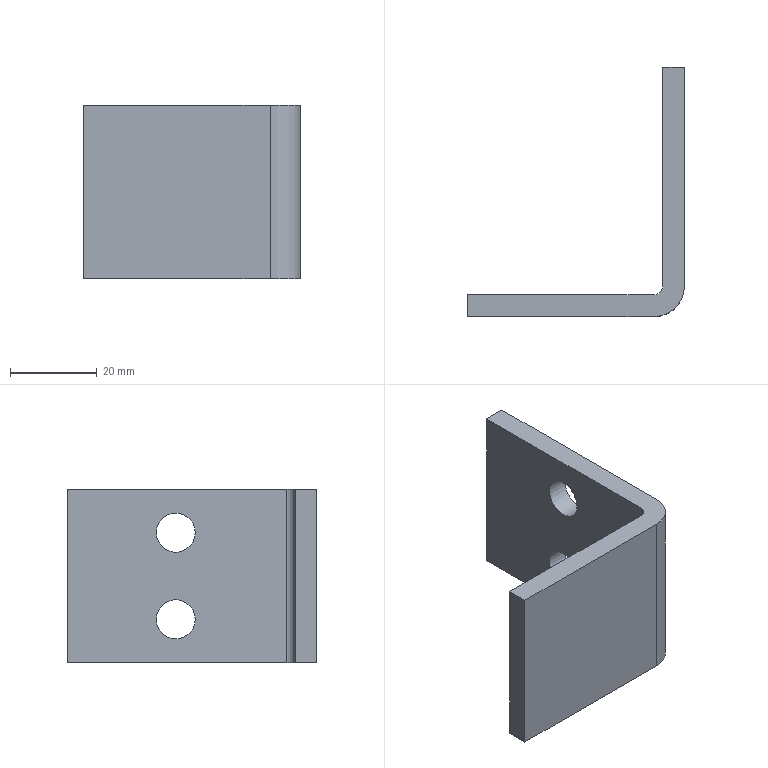Component | NX | CH3404_2-4 | 1 solid | 12 faces | box 50 x 57.5 x 40 mm | volume 19478 mm3 | plane 8 | cylinder 4 | commonest cylinder face diameters 9 x2 4 x1 14 x1
STEP:
#1=CARTESIAN_POINT('',(0.,0.,0.));
#2=DIRECTION('',(0.,0.,1.));
#3=DIRECTION('',(1.,0.,0.));
#4=AXIS2_PLACEMENT_3D('',#1,#2,#3);
#5=CARTESIAN_POINT('',(-0.,25.5,10.));
#6=VERTEX_POINT('',#5);
#7=CARTESIAN_POINT('',(0.,34.5,10.));
#8=VERTEX_POINT('',#7);
#9=CARTESIAN_POINT('',(-0.,30.,10.));
#10=DIRECTION('',(-1.,-0.,0.));
#11=DIRECTION('',(0.,-1.,0.));
#12=AXIS2_PLACEMENT_3D('',#9,#10,#11);
#13=CIRCLE('',#12,4.5);
#14=CARTESIAN_POINT('',(0.,-2.5,20.));
#15=DIRECTION('',(-1.,-0.,0.));
#16=DIRECTION('',(0.,-1.,0.));
#17=AXIS2_PLACEMENT_3D('',#14,#15,#16);
#18=PLANE('',#17);
#19=CARTESIAN_POINT('',(-32.5,-10.));
#20=DIRECTION('',(1.,0.));
#21=AXIS2_PLACEMENT_2D('',#19,#20);
#22=CIRCLE('',#21,4.5);
#23=(GEOMETRIC_REPRESENTATION_CONTEXT(2)PARAMETRIC_REPRESENTATION_CONTEXT()REPRESENTATION_CONTEXT('',''));
#24=DEFINITIONAL_REPRESENTATION('',(#22),#23);
#25=PCURVE('',#18,#24);
#26=CARTESIAN_POINT('',(-5.,30.,10.));
#27=DIRECTION('',(1.,-0.,0.));
#28=DIRECTION('',(0.,1.,0.));
#29=AXIS2_PLACEMENT_3D('',#26,#27,#28);
#30=CYLINDRICAL_SURFACE('',#29,4.5);
#31=CARTESIAN_POINT('',(3.142,5.));
#32=DIRECTION('',(-1.,0.));
#33=VECTOR('',#32,1.);
#34=LINE('',#31,#33);
#35=(GEOMETRIC_REPRESENTATION_CONTEXT(2)PARAMETRIC_REPRESENTATION_CONTEXT()REPRESENTATION_CONTEXT('',''));
#36=DEFINITIONAL_REPRESENTATION('',(#34),#35);
#37=PCURVE('',#30,#36);
#38=SURFACE_CURVE('',#13,(#25,#37),.PCURVE_S1.);
#39=EDGE_CURVE('',#6,#8,#38,.T.);
#40=ORIENTED_EDGE('',*,*,#39,.T.);
#41=CARTESIAN_POINT('',(-0.,30.,10.));
#42=DIRECTION('',(-1.,-0.,0.));
#43=DIRECTION('',(0.,-1.,0.));
#44=AXIS2_PLACEMENT_3D('',#41,#42,#43);
#45=CIRCLE('',#44,4.5);
#46=CARTESIAN_POINT('',(-32.5,-10.));
#47=DIRECTION('',(1.,0.));
#48=AXIS2_PLACEMENT_2D('',#46,#47);
#49=CIRCLE('',#48,4.5);
#50=(GEOMETRIC_REPRESENTATION_CONTEXT(2)PARAMETRIC_REPRESENTATION_CONTEXT()REPRESENTATION_CONTEXT('',''));
#51=DEFINITIONAL_REPRESENTATION('',(#49),#50);
#52=PCURVE('',#18,#51);
#53=CARTESIAN_POINT('',(9.425,5.));
#54=DIRECTION('',(-1.,0.));
#55=VECTOR('',#54,1.);
#56=LINE('',#53,#55);
#57=(GEOMETRIC_REPRESENTATION_CONTEXT(2)PARAMETRIC_REPRESENTATION_CONTEXT()REPRESENTATION_CONTEXT('',''));
#58=DEFINITIONAL_REPRESENTATION('',(#56),#57);
#59=PCURVE('',#30,#58);
#60=SURFACE_CURVE('',#45,(#52,#59),.PCURVE_S1.);
#61=EDGE_CURVE('',#8,#6,#60,.T.);
#62=ORIENTED_EDGE('',*,*,#61,.T.);
#63=EDGE_LOOP('',(#40,#62));
#64=FACE_BOUND('',#63,.T.);
#65=CARTESIAN_POINT('',(-0.,25.5,-10.));
#66=VERTEX_POINT('',#65);
#67=CARTESIAN_POINT('',(0.,34.5,-10.));
#68=VERTEX_POINT('',#67);
#69=CARTESIAN_POINT('',(-0.,30.,-10.));
#70=DIRECTION('',(-1.,-0.,0.));
#71=DIRECTION('',(0.,-1.,0.));
#72=AXIS2_PLACEMENT_3D('',#69,#70,#71);
#73=CIRCLE('',#72,4.5);
#74=CARTESIAN_POINT('',(-32.5,-30.));
#75=DIRECTION('',(1.,0.));
#76=AXIS2_PLACEMENT_2D('',#74,#75);
#77=CIRCLE('',#76,4.5);
#78=(GEOMETRIC_REPRESENTATION_CONTEXT(2)PARAMETRIC_REPRESENTATION_CONTEXT()REPRESENTATION_CONTEXT('',''));
#79=DEFINITIONAL_REPRESENTATION('',(#77),#78);
#80=PCURVE('',#18,#79);
#81=CARTESIAN_POINT('',(-5.,30.,-10.));
#82=DIRECTION('',(1.,-0.,0.));
#83=DIRECTION('',(0.,1.,0.));
#84=AXIS2_PLACEMENT_3D('',#81,#82,#83);
#85=CYLINDRICAL_SURFACE('',#84,4.5);
#86=CARTESIAN_POINT('',(3.142,5.));
#87=DIRECTION('',(-1.,0.));
#88=VECTOR('',#87,1.);
#89=LINE('',#86,#88);
#90=(GEOMETRIC_REPRESENTATION_CONTEXT(2)PARAMETRIC_REPRESENTATION_CONTEXT()REPRESENTATION_CONTEXT('',''));
#91=DEFINITIONAL_REPRESENTATION('',(#89),#90);
#92=PCURVE('',#85,#91);
#93=SURFACE_CURVE('',#73,(#80,#92),.PCURVE_S1.);
#94=EDGE_CURVE('',#66,#68,#93,.T.);
#95=ORIENTED_EDGE('',*,*,#94,.T.);
#96=CARTESIAN_POINT('',(-0.,30.,-10.));
#97=DIRECTION('',(-1.,-0.,0.));
#98=DIRECTION('',(0.,-1.,0.));
#99=AXIS2_PLACEMENT_3D('',#96,#97,#98);
#100=CIRCLE('',#99,4.5);
#101=CARTESIAN_POINT('',(-32.5,-30.));
#102=DIRECTION('',(1.,0.));
#103=AXIS2_PLACEMENT_2D('',#101,#102);
#104=CIRCLE('',#103,4.5);
#105=(GEOMETRIC_REPRESENTATION_CONTEXT(2)PARAMETRIC_REPRESENTATION_CONTEXT()REPRESENTATION_CONTEXT('',''));
#106=DEFINITIONAL_REPRESENTATION('',(#104),#105);
#107=PCURVE('',#18,#106);
#108=CARTESIAN_POINT('',(9.425,5.));
#109=DIRECTION('',(-1.,0.));
#110=VECTOR('',#109,1.);
#111=LINE('',#108,#110);
#112=(GEOMETRIC_REPRESENTATION_CONTEXT(2)PARAMETRIC_REPRESENTATION_CONTEXT()REPRESENTATION_CONTEXT('',''));
#113=DEFINITIONAL_REPRESENTATION('',(#111),#112);
#114=PCURVE('',#85,#113);
#115=SURFACE_CURVE('',#100,(#107,#114),.PCURVE_S1.);
#116=EDGE_CURVE('',#68,#66,#115,.T.);
#117=ORIENTED_EDGE('',*,*,#116,.T.);
#118=EDGE_LOOP('',(#95,#117));
#119=FACE_BOUND('',#118,.T.);
#120=CARTESIAN_POINT('',(0.,4.5,20.));
#121=VERTEX_POINT('',#120);
#122=CARTESIAN_POINT('',(-0.,55.,20.));
#123=VERTEX_POINT('',#122);
#124=CARTESIAN_POINT('',(0.,-2.5,20.));
#125=DIRECTION('',(-0.,1.,0.));
#126=VECTOR('',#125,1.);
#127=LINE('',#124,#126);
#128=CARTESIAN_POINT('',(0.,0.));
#129=DIRECTION('',(-1.,0.));
#130=VECTOR('',#129,1.);
#131=LINE('',#128,#130);
#132=(GEOMETRIC_REPRESENTATION_CONTEXT(2)PARAMETRIC_REPRESENTATION_CONTEXT()REPRESENTATION_CONTEXT('',''));
#133=DEFINITIONAL_REPRESENTATION('',(#131),#132);
#134=PCURVE('',#18,#133);
#135=CARTESIAN_POINT('',(0.,0.,20.));
#136=DIRECTION('',(0.,0.,1.));
#137=DIRECTION('',(1.,0.,0.));
#138=AXIS2_PLACEMENT_3D('',#135,#136,#137);
#139=PLANE('',#138);
#140=CARTESIAN_POINT('',(0.,-2.5));
#141=DIRECTION('',(-0.,1.));
#142=VECTOR('',#141,1.);
#143=LINE('',#140,#142);
#144=(GEOMETRIC_REPRESENTATION_CONTEXT(2)PARAMETRIC_REPRESENTATION_CONTEXT()REPRESENTATION_CONTEXT('',''));
#145=DEFINITIONAL_REPRESENTATION('',(#143),#144);
#146=PCURVE('',#139,#145);
#147=SURFACE_CURVE('',#127,(#134,#146),.PCURVE_S1.);
#148=EDGE_CURVE('',#121,#123,#147,.T.);
#149=ORIENTED_EDGE('',*,*,#148,.F.);
#150=CARTESIAN_POINT('',(0.,4.5,-20.));
#151=VERTEX_POINT('',#150);
#152=CARTESIAN_POINT('',(0.,4.5,20.));
#153=DIRECTION('',(0.,0.,-1.));
#154=VECTOR('',#153,1.);
#155=LINE('',#152,#154);
#156=CARTESIAN_POINT('',(-7.,0.));
#157=DIRECTION('',(0.,-1.));
#158=VECTOR('',#157,1.);
#159=LINE('',#156,#158);
#160=(GEOMETRIC_REPRESENTATION_CONTEXT(2)PARAMETRIC_REPRESENTATION_CONTEXT()REPRESENTATION_CONTEXT('',''));
#161=DEFINITIONAL_REPRESENTATION('',(#159),#160);
#162=PCURVE('',#18,#161);
#163=CARTESIAN_POINT('',(-7.,4.5,20.));
#164=DIRECTION('',(0.,0.,-1.));
#165=DIRECTION('',(-1.,0.,0.));
#166=AXIS2_PLACEMENT_3D('',#163,#164,#165);
#167=CYLINDRICAL_SURFACE('',#166,7.);
#168=CARTESIAN_POINT('',(3.142,0.));
#169=DIRECTION('',(0.,1.));
#170=VECTOR('',#169,1.);
#171=LINE('',#168,#170);
#172=(GEOMETRIC_REPRESENTATION_CONTEXT(2)PARAMETRIC_REPRESENTATION_CONTEXT()REPRESENTATION_CONTEXT('',''));
#173=DEFINITIONAL_REPRESENTATION('',(#171),#172);
#174=PCURVE('',#167,#173);
#175=SURFACE_CURVE('',#155,(#162,#174),.PCURVE_S1.);
#176=EDGE_CURVE('',#121,#151,#175,.T.);
#177=ORIENTED_EDGE('',*,*,#176,.T.);
#178=CARTESIAN_POINT('',(-0.,55.,-20.));
#179=VERTEX_POINT('',#178);
#180=CARTESIAN_POINT('',(0.,-2.5,-20.));
#181=DIRECTION('',(-0.,1.,0.));
#182=VECTOR('',#181,1.);
#183=LINE('',#180,#182);
#184=CARTESIAN_POINT('',(0.,-40.));
#185=DIRECTION('',(-1.,0.));
#186=VECTOR('',#185,1.);
#187=LINE('',#184,#186);
#188=(GEOMETRIC_REPRESENTATION_CONTEXT(2)PARAMETRIC_REPRESENTATION_CONTEXT()REPRESENTATION_CONTEXT('',''));
#189=DEFINITIONAL_REPRESENTATION('',(#187),#188);
#190=PCURVE('',#18,#189);
#191=CARTESIAN_POINT('',(0.,0.,-20.));
#192=DIRECTION('',(0.,0.,1.));
#193=DIRECTION('',(1.,0.,0.));
#194=AXIS2_PLACEMENT_3D('',#191,#192,#193);
#195=PLANE('',#194);
#196=CARTESIAN_POINT('',(0.,-2.5));
#197=DIRECTION('',(-0.,1.));
#198=VECTOR('',#197,1.);
#199=LINE('',#196,#198);
#200=(GEOMETRIC_REPRESENTATION_CONTEXT(2)PARAMETRIC_REPRESENTATION_CONTEXT()REPRESENTATION_CONTEXT('',''));
#201=DEFINITIONAL_REPRESENTATION('',(#199),#200);
#202=PCURVE('',#195,#201);
#203=SURFACE_CURVE('',#183,(#190,#202),.PCURVE_S1.);
#204=EDGE_CURVE('',#151,#179,#203,.T.);
#205=ORIENTED_EDGE('',*,*,#204,.T.);
#206=CARTESIAN_POINT('',(-0.,55.,20.));
#207=DIRECTION('',(0.,0.,-1.));
#208=VECTOR('',#207,1.);
#209=LINE('',#206,#208);
#210=CARTESIAN_POINT('',(-57.5,0.));
#211=DIRECTION('',(0.,-1.));
#212=VECTOR('',#211,1.);
#213=LINE('',#210,#212);
#214=(GEOMETRIC_REPRESENTATION_CONTEXT(2)PARAMETRIC_REPRESENTATION_CONTEXT()REPRESENTATION_CONTEXT('',''));
#215=DEFINITIONAL_REPRESENTATION('',(#213),#214);
#216=PCURVE('',#18,#215);
#217=CARTESIAN_POINT('',(-0.,55.,20.));
#218=DIRECTION('',(0.,-1.,0.));
#219=DIRECTION('',(1.,0.,0.));
#220=AXIS2_PLACEMENT_3D('',#217,#218,#219);
#221=PLANE('',#220);
#222=CARTESIAN_POINT('',(0.,0.));
#223=DIRECTION('',(0.,-1.));
#224=VECTOR('',#223,1.);
#225=LINE('',#222,#224);
#226=(GEOMETRIC_REPRESENTATION_CONTEXT(2)PARAMETRIC_REPRESENTATION_CONTEXT()REPRESENTATION_CONTEXT('',''));
#227=DEFINITIONAL_REPRESENTATION('',(#225),#226);
#228=PCURVE('',#221,#227);
#229=SURFACE_CURVE('',#209,(#216,#228),.PCURVE_S1.);
#230=EDGE_CURVE('',#123,#179,#229,.T.);
#231=ORIENTED_EDGE('',*,*,#230,.F.);
#232=EDGE_LOOP('',(#149,#177,#205,#231));
#233=FACE_BOUND('',#232,.T.);
#234=ADVANCED_FACE('',(#64,#119,#233),#18,.F.);
#235=CARTESIAN_POINT('',(-5.,55.,-20.));
#236=VERTEX_POINT('',#235);
#237=CARTESIAN_POINT('',(-0.,55.,-20.));
#238=DIRECTION('',(-1.,0.,0.));
#239=VECTOR('',#238,1.);
#240=LINE('',#237,#239);
#241=CARTESIAN_POINT('',(0.,-40.));
#242=DIRECTION('',(-1.,0.));
#243=VECTOR('',#242,1.);
#244=LINE('',#241,#243);
#245=(GEOMETRIC_REPRESENTATION_CONTEXT(2)PARAMETRIC_REPRESENTATION_CONTEXT()REPRESENTATION_CONTEXT('',''));
#246=DEFINITIONAL_REPRESENTATION('',(#244),#245);
#247=PCURVE('',#221,#246);
#248=CARTESIAN_POINT('',(-0.,55.));
#249=DIRECTION('',(-1.,0.));
#250=VECTOR('',#249,1.);
#251=LINE('',#248,#250);
#252=(GEOMETRIC_REPRESENTATION_CONTEXT(2)PARAMETRIC_REPRESENTATION_CONTEXT()REPRESENTATION_CONTEXT('',''));
#253=DEFINITIONAL_REPRESENTATION('',(#251),#252);
#254=PCURVE('',#195,#253);
#255=SURFACE_CURVE('',#240,(#247,#254),.PCURVE_S1.);
#256=EDGE_CURVE('',#179,#236,#255,.T.);
#257=ORIENTED_EDGE('',*,*,#256,.T.);
#258=CARTESIAN_POINT('',(-5.,55.,20.));
#259=VERTEX_POINT('',#258);
#260=CARTESIAN_POINT('',(-5.,55.,20.));
#261=DIRECTION('',(0.,0.,-1.));
#262=VECTOR('',#261,1.);
#263=LINE('',#260,#262);
#264=CARTESIAN_POINT('',(-5.,0.));
#265=DIRECTION('',(0.,-1.));
#266=VECTOR('',#265,1.);
#267=LINE('',#264,#266);
#268=(GEOMETRIC_REPRESENTATION_CONTEXT(2)PARAMETRIC_REPRESENTATION_CONTEXT()REPRESENTATION_CONTEXT('',''));
#269=DEFINITIONAL_REPRESENTATION('',(#267),#268);
#270=PCURVE('',#221,#269);
#271=CARTESIAN_POINT('',(-5.,55.,20.));
#272=DIRECTION('',(1.,0.,0.));
#273=DIRECTION('',(0.,0.,-1.));
#274=AXIS2_PLACEMENT_3D('',#271,#272,#273);
#275=PLANE('',#274);
#276=CARTESIAN_POINT('',(0.,0.));
#277=DIRECTION('',(1.,0.));
#278=VECTOR('',#277,1.);
#279=LINE('',#276,#278);
#280=(GEOMETRIC_REPRESENTATION_CONTEXT(2)PARAMETRIC_REPRESENTATION_CONTEXT()REPRESENTATION_CONTEXT('',''));
#281=DEFINITIONAL_REPRESENTATION('',(#279),#280);
#282=PCURVE('',#275,#281);
#283=SURFACE_CURVE('',#263,(#270,#282),.PCURVE_S1.);
#284=EDGE_CURVE('',#259,#236,#283,.T.);
#285=ORIENTED_EDGE('',*,*,#284,.F.);
#286=CARTESIAN_POINT('',(-0.,55.,20.));
#287=DIRECTION('',(-1.,0.,0.));
#288=VECTOR('',#287,1.);
#289=LINE('',#286,#288);
#290=CARTESIAN_POINT('',(0.,0.));
#291=DIRECTION('',(-1.,0.));
#292=VECTOR('',#291,1.);
#293=LINE('',#290,#292);
#294=(GEOMETRIC_REPRESENTATION_CONTEXT(2)PARAMETRIC_REPRESENTATION_CONTEXT()REPRESENTATION_CONTEXT('',''));
#295=DEFINITIONAL_REPRESENTATION('',(#293),#294);
#296=PCURVE('',#221,#295);
#297=CARTESIAN_POINT('',(-0.,55.));
#298=DIRECTION('',(-1.,0.));
#299=VECTOR('',#298,1.);
#300=LINE('',#297,#299);
#301=(GEOMETRIC_REPRESENTATION_CONTEXT(2)PARAMETRIC_REPRESENTATION_CONTEXT()REPRESENTATION_CONTEXT('',''));
#302=DEFINITIONAL_REPRESENTATION('',(#300),#301);
#303=PCURVE('',#139,#302);
#304=SURFACE_CURVE('',#289,(#296,#303),.PCURVE_S1.);
#305=EDGE_CURVE('',#123,#259,#304,.T.);
#306=ORIENTED_EDGE('',*,*,#305,.F.);
#307=ORIENTED_EDGE('',*,*,#230,.T.);
#308=EDGE_LOOP('',(#257,#285,#306,#307));
#309=FACE_BOUND('',#308,.T.);
#310=ADVANCED_FACE('',(#309),#221,.F.);
#311=CARTESIAN_POINT('',(-5.,34.5,10.));
#312=VERTEX_POINT('',#311);
#313=CARTESIAN_POINT('',(-5.,30.,10.));
#314=DIRECTION('',(1.,-0.,0.));
#315=DIRECTION('',(0.,1.,0.));
#316=AXIS2_PLACEMENT_3D('',#313,#314,#315);
#317=CIRCLE('',#316,4.5);
#318=CARTESIAN_POINT('',(10.,-25.));
#319=DIRECTION('',(0.,1.));
#320=AXIS2_PLACEMENT_2D('',#318,#319);
#321=CIRCLE('',#320,4.5);
#322=(GEOMETRIC_REPRESENTATION_CONTEXT(2)PARAMETRIC_REPRESENTATION_CONTEXT()REPRESENTATION_CONTEXT('',''));
#323=DEFINITIONAL_REPRESENTATION('',(#321),#322);
#324=PCURVE('',#275,#323);
#325=CARTESIAN_POINT('',(0.,0.));
#326=DIRECTION('',(1.,0.));
#327=VECTOR('',#326,1.);
#328=LINE('',#325,#327);
#329=(GEOMETRIC_REPRESENTATION_CONTEXT(2)PARAMETRIC_REPRESENTATION_CONTEXT()REPRESENTATION_CONTEXT('',''));
#330=DEFINITIONAL_REPRESENTATION('',(#328),#329);
#331=PCURVE('',#30,#330);
#332=SURFACE_CURVE('',#317,(#324,#331),.PCURVE_S1.);
#333=EDGE_CURVE('',#312,#312,#332,.T.);
#334=ORIENTED_EDGE('',*,*,#333,.T.);
#335=EDGE_LOOP('',(#334));
#336=FACE_BOUND('',#335,.T.);
#337=CARTESIAN_POINT('',(-5.,34.5,-10.));
#338=VERTEX_POINT('',#337);
#339=CARTESIAN_POINT('',(-5.,30.,-10.));
#340=DIRECTION('',(1.,-0.,0.));
#341=DIRECTION('',(0.,1.,0.));
#342=AXIS2_PLACEMENT_3D('',#339,#340,#341);
#343=CIRCLE('',#342,4.5);
#344=CARTESIAN_POINT('',(30.,-25.));
#345=DIRECTION('',(0.,1.));
#346=AXIS2_PLACEMENT_2D('',#344,#345);
#347=CIRCLE('',#346,4.5);
#348=(GEOMETRIC_REPRESENTATION_CONTEXT(2)PARAMETRIC_REPRESENTATION_CONTEXT()REPRESENTATION_CONTEXT('',''));
#349=DEFINITIONAL_REPRESENTATION('',(#347),#348);
#350=PCURVE('',#275,#349);
#351=CARTESIAN_POINT('',(0.,0.));
#352=DIRECTION('',(1.,0.));
#353=VECTOR('',#352,1.);
#354=LINE('',#351,#353);
#355=(GEOMETRIC_REPRESENTATION_CONTEXT(2)PARAMETRIC_REPRESENTATION_CONTEXT()REPRESENTATION_CONTEXT('',''));
#356=DEFINITIONAL_REPRESENTATION('',(#354),#355);
#357=PCURVE('',#85,#356);
#358=SURFACE_CURVE('',#343,(#350,#357),.PCURVE_S1.);
#359=EDGE_CURVE('',#338,#338,#358,.T.);
#360=ORIENTED_EDGE('',*,*,#359,.T.);
#361=EDGE_LOOP('',(#360));
#362=FACE_BOUND('',#361,.T.);
#363=CARTESIAN_POINT('',(-5.,4.5,-20.));
#364=VERTEX_POINT('',#363);
#365=CARTESIAN_POINT('',(-5.,55.,-20.));
#366=DIRECTION('',(0.,-1.,0.));
#367=VECTOR('',#366,1.);
#368=LINE('',#365,#367);
#369=CARTESIAN_POINT('',(40.,0.));
#370=DIRECTION('',(0.,-1.));
#371=VECTOR('',#370,1.);
#372=LINE('',#369,#371);
#373=(GEOMETRIC_REPRESENTATION_CONTEXT(2)PARAMETRIC_REPRESENTATION_CONTEXT()REPRESENTATION_CONTEXT('',''));
#374=DEFINITIONAL_REPRESENTATION('',(#372),#373);
#375=PCURVE('',#275,#374);
#376=CARTESIAN_POINT('',(-5.,55.));
#377=DIRECTION('',(0.,-1.));
#378=VECTOR('',#377,1.);
#379=LINE('',#376,#378);
#380=(GEOMETRIC_REPRESENTATION_CONTEXT(2)PARAMETRIC_REPRESENTATION_CONTEXT()REPRESENTATION_CONTEXT('',''));
#381=DEFINITIONAL_REPRESENTATION('',(#379),#380);
#382=PCURVE('',#195,#381);
#383=SURFACE_CURVE('',#368,(#375,#382),.PCURVE_S1.);
#384=EDGE_CURVE('',#236,#364,#383,.T.);
#385=ORIENTED_EDGE('',*,*,#384,.T.);
#386=CARTESIAN_POINT('',(-5.,4.5,20.));
#387=VERTEX_POINT('',#386);
#388=CARTESIAN_POINT('',(-5.,4.5,20.));
#389=DIRECTION('',(0.,0.,1.));
#390=VECTOR('',#389,1.);
#391=LINE('',#388,#390);
#392=CARTESIAN_POINT('',(0.,-50.5));
#393=DIRECTION('',(-1.,0.));
#394=VECTOR('',#393,1.);
#395=LINE('',#392,#394);
#396=(GEOMETRIC_REPRESENTATION_CONTEXT(2)PARAMETRIC_REPRESENTATION_CONTEXT()REPRESENTATION_CONTEXT('',''));
#397=DEFINITIONAL_REPRESENTATION('',(#395),#396);
#398=PCURVE('',#275,#397);
#399=CARTESIAN_POINT('',(-7.,4.5,20.));
#400=DIRECTION('',(0.,0.,1.));
#401=DIRECTION('',(1.,0.,0.));
#402=AXIS2_PLACEMENT_3D('',#399,#400,#401);
#403=CYLINDRICAL_SURFACE('',#402,2.);
#404=CARTESIAN_POINT('',(6.283,0.));
#405=DIRECTION('',(0.,1.));
#406=VECTOR('',#405,1.);
#407=LINE('',#404,#406);
#408=(GEOMETRIC_REPRESENTATION_CONTEXT(2)PARAMETRIC_REPRESENTATION_CONTEXT()REPRESENTATION_CONTEXT('',''));
#409=DEFINITIONAL_REPRESENTATION('',(#407),#408);
#410=PCURVE('',#403,#409);
#411=SURFACE_CURVE('',#391,(#398,#410),.PCURVE_S1.);
#412=EDGE_CURVE('',#364,#387,#411,.T.);
#413=ORIENTED_EDGE('',*,*,#412,.T.);
#414=CARTESIAN_POINT('',(-5.,55.,20.));
#415=DIRECTION('',(0.,-1.,0.));
#416=VECTOR('',#415,1.);
#417=LINE('',#414,#416);
#418=CARTESIAN_POINT('',(0.,0.));
#419=DIRECTION('',(0.,-1.));
#420=VECTOR('',#419,1.);
#421=LINE('',#418,#420);
#422=(GEOMETRIC_REPRESENTATION_CONTEXT(2)PARAMETRIC_REPRESENTATION_CONTEXT()REPRESENTATION_CONTEXT('',''));
#423=DEFINITIONAL_REPRESENTATION('',(#421),#422);
#424=PCURVE('',#275,#423);
#425=CARTESIAN_POINT('',(-5.,55.));
#426=DIRECTION('',(0.,-1.));
#427=VECTOR('',#426,1.);
#428=LINE('',#425,#427);
#429=(GEOMETRIC_REPRESENTATION_CONTEXT(2)PARAMETRIC_REPRESENTATION_CONTEXT()REPRESENTATION_CONTEXT('',''));
#430=DEFINITIONAL_REPRESENTATION('',(#428),#429);
#431=PCURVE('',#139,#430);
#432=SURFACE_CURVE('',#417,(#424,#431),.PCURVE_S1.);
#433=EDGE_CURVE('',#259,#387,#432,.T.);
#434=ORIENTED_EDGE('',*,*,#433,.F.);
#435=ORIENTED_EDGE('',*,*,#284,.T.);
#436=EDGE_LOOP('',(#385,#413,#434,#435));
#437=FACE_BOUND('',#436,.T.);
#438=ADVANCED_FACE('',(#336,#362,#437),#275,.F.);
#439=CARTESIAN_POINT('',(-7.,2.5,20.));
#440=VERTEX_POINT('',#439);
#441=CARTESIAN_POINT('',(-50.,2.5,20.));
#442=VERTEX_POINT('',#441);
#443=CARTESIAN_POINT('',(-5.,2.5,20.));
#444=DIRECTION('',(-1.,-0.,0.));
#445=VECTOR('',#444,1.);
#446=LINE('',#443,#445);
#447=CARTESIAN_POINT('',(-5.,2.5,20.));
#448=DIRECTION('',(0.,-1.,0.));
#449=DIRECTION('',(1.,0.,0.));
#450=AXIS2_PLACEMENT_3D('',#447,#448,#449);
#451=PLANE('',#450);
#452=CARTESIAN_POINT('',(0.,0.));
#453=DIRECTION('',(-1.,0.));
#454=VECTOR('',#453,1.);
#455=LINE('',#452,#454);
#456=(GEOMETRIC_REPRESENTATION_CONTEXT(2)PARAMETRIC_REPRESENTATION_CONTEXT()REPRESENTATION_CONTEXT('',''));
#457=DEFINITIONAL_REPRESENTATION('',(#455),#456);
#458=PCURVE('',#451,#457);
#459=CARTESIAN_POINT('',(-5.,2.5));
#460=DIRECTION('',(-1.,-0.));
#461=VECTOR('',#460,1.);
#462=LINE('',#459,#461);
#463=(GEOMETRIC_REPRESENTATION_CONTEXT(2)PARAMETRIC_REPRESENTATION_CONTEXT()REPRESENTATION_CONTEXT('',''));
#464=DEFINITIONAL_REPRESENTATION('',(#462),#463);
#465=PCURVE('',#139,#464);
#466=SURFACE_CURVE('',#446,(#458,#465),.PCURVE_S1.);
#467=EDGE_CURVE('',#440,#442,#466,.T.);
#468=ORIENTED_EDGE('',*,*,#467,.F.);
#469=CARTESIAN_POINT('',(-7.,2.5,-20.));
#470=VERTEX_POINT('',#469);
#471=CARTESIAN_POINT('',(-7.,2.5,-20.));
#472=DIRECTION('',(0.,0.,-1.));
#473=VECTOR('',#472,1.);
#474=LINE('',#471,#473);
#475=CARTESIAN_POINT('',(-2.,-40.));
#476=DIRECTION('',(0.,-1.));
#477=VECTOR('',#476,1.);
#478=LINE('',#475,#477);
#479=(GEOMETRIC_REPRESENTATION_CONTEXT(2)PARAMETRIC_REPRESENTATION_CONTEXT()REPRESENTATION_CONTEXT('',''));
#480=DEFINITIONAL_REPRESENTATION('',(#478),#479);
#481=PCURVE('',#451,#480);
#482=CARTESIAN_POINT('',(4.712,-40.));
#483=DIRECTION('',(0.,-1.));
#484=VECTOR('',#483,1.);
#485=LINE('',#482,#484);
#486=(GEOMETRIC_REPRESENTATION_CONTEXT(2)PARAMETRIC_REPRESENTATION_CONTEXT()REPRESENTATION_CONTEXT('',''));
#487=DEFINITIONAL_REPRESENTATION('',(#485),#486);
#488=PCURVE('',#403,#487);
#489=SURFACE_CURVE('',#474,(#481,#488),.PCURVE_S1.);
#490=EDGE_CURVE('',#440,#470,#489,.T.);
#491=ORIENTED_EDGE('',*,*,#490,.T.);
#492=CARTESIAN_POINT('',(-50.,2.5,-20.));
#493=VERTEX_POINT('',#492);
#494=CARTESIAN_POINT('',(-5.,2.5,-20.));
#495=DIRECTION('',(-1.,-0.,0.));
#496=VECTOR('',#495,1.);
#497=LINE('',#494,#496);
#498=CARTESIAN_POINT('',(0.,-40.));
#499=DIRECTION('',(-1.,0.));
#500=VECTOR('',#499,1.);
#501=LINE('',#498,#500);
#502=(GEOMETRIC_REPRESENTATION_CONTEXT(2)PARAMETRIC_REPRESENTATION_CONTEXT()REPRESENTATION_CONTEXT('',''));
#503=DEFINITIONAL_REPRESENTATION('',(#501),#502);
#504=PCURVE('',#451,#503);
#505=CARTESIAN_POINT('',(-5.,2.5));
#506=DIRECTION('',(-1.,-0.));
#507=VECTOR('',#506,1.);
#508=LINE('',#505,#507);
#509=(GEOMETRIC_REPRESENTATION_CONTEXT(2)PARAMETRIC_REPRESENTATION_CONTEXT()REPRESENTATION_CONTEXT('',''));
#510=DEFINITIONAL_REPRESENTATION('',(#508),#509);
#511=PCURVE('',#195,#510);
#512=SURFACE_CURVE('',#497,(#504,#511),.PCURVE_S1.);
#513=EDGE_CURVE('',#470,#493,#512,.T.);
#514=ORIENTED_EDGE('',*,*,#513,.T.);
#515=CARTESIAN_POINT('',(-50.,2.5,20.));
#516=DIRECTION('',(0.,0.,-1.));
#517=VECTOR('',#516,1.);
#518=LINE('',#515,#517);
#519=CARTESIAN_POINT('',(-45.,0.));
#520=DIRECTION('',(0.,-1.));
#521=VECTOR('',#520,1.);
#522=LINE('',#519,#521);
#523=(GEOMETRIC_REPRESENTATION_CONTEXT(2)PARAMETRIC_REPRESENTATION_CONTEXT()REPRESENTATION_CONTEXT('',''));
#524=DEFINITIONAL_REPRESENTATION('',(#522),#523);
#525=PCURVE('',#451,#524);
#526=CARTESIAN_POINT('',(-50.,2.5,20.));
#527=DIRECTION('',(1.,0.,0.));
#528=DIRECTION('',(0.,0.,-1.));
#529=AXIS2_PLACEMENT_3D('',#526,#527,#528);
#530=PLANE('',#529);
#531=CARTESIAN_POINT('',(0.,0.));
#532=DIRECTION('',(1.,0.));
#533=VECTOR('',#532,1.);
#534=LINE('',#531,#533);
#535=(GEOMETRIC_REPRESENTATION_CONTEXT(2)PARAMETRIC_REPRESENTATION_CONTEXT()REPRESENTATION_CONTEXT('',''));
#536=DEFINITIONAL_REPRESENTATION('',(#534),#535);
#537=PCURVE('',#530,#536);
#538=SURFACE_CURVE('',#518,(#525,#537),.PCURVE_S1.);
#539=EDGE_CURVE('',#442,#493,#538,.T.);
#540=ORIENTED_EDGE('',*,*,#539,.F.);
#541=EDGE_LOOP('',(#468,#491,#514,#540));
#542=FACE_BOUND('',#541,.T.);
#543=ADVANCED_FACE('',(#542),#451,.F.);
#544=CARTESIAN_POINT('',(-50.,-2.5,-20.));
#545=VERTEX_POINT('',#544);
#546=CARTESIAN_POINT('',(-50.,2.5,-20.));
#547=DIRECTION('',(0.,-1.,0.));
#548=VECTOR('',#547,1.);
#549=LINE('',#546,#548);
#550=CARTESIAN_POINT('',(40.,0.));
#551=DIRECTION('',(0.,-1.));
#552=VECTOR('',#551,1.);
#553=LINE('',#550,#552);
#554=(GEOMETRIC_REPRESENTATION_CONTEXT(2)PARAMETRIC_REPRESENTATION_CONTEXT()REPRESENTATION_CONTEXT('',''));
#555=DEFINITIONAL_REPRESENTATION('',(#553),#554);
#556=PCURVE('',#530,#555);
#557=CARTESIAN_POINT('',(-50.,2.5));
#558=DIRECTION('',(0.,-1.));
#559=VECTOR('',#558,1.);
#560=LINE('',#557,#559);
#561=(GEOMETRIC_REPRESENTATION_CONTEXT(2)PARAMETRIC_REPRESENTATION_CONTEXT()REPRESENTATION_CONTEXT('',''));
#562=DEFINITIONAL_REPRESENTATION('',(#560),#561);
#563=PCURVE('',#195,#562);
#564=SURFACE_CURVE('',#549,(#556,#563),.PCURVE_S1.);
#565=EDGE_CURVE('',#493,#545,#564,.T.);
#566=ORIENTED_EDGE('',*,*,#565,.T.);
#567=CARTESIAN_POINT('',(-50.,-2.5,20.));
#568=VERTEX_POINT('',#567);
#569=CARTESIAN_POINT('',(-50.,-2.5,20.));
#570=DIRECTION('',(0.,0.,-1.));
#571=VECTOR('',#570,1.);
#572=LINE('',#569,#571);
#573=CARTESIAN_POINT('',(0.,-5.));
#574=DIRECTION('',(1.,0.));
#575=VECTOR('',#574,1.);
#576=LINE('',#573,#575);
#577=(GEOMETRIC_REPRESENTATION_CONTEXT(2)PARAMETRIC_REPRESENTATION_CONTEXT()REPRESENTATION_CONTEXT('',''));
#578=DEFINITIONAL_REPRESENTATION('',(#576),#577);
#579=PCURVE('',#530,#578);
#580=CARTESIAN_POINT('',(-50.,-2.5,20.));
#581=DIRECTION('',(-0.,1.,0.));
#582=DIRECTION('',(-1.,-0.,0.));
#583=AXIS2_PLACEMENT_3D('',#580,#581,#582);
#584=PLANE('',#583);
#585=CARTESIAN_POINT('',(0.,0.));
#586=DIRECTION('',(0.,-1.));
#587=VECTOR('',#586,1.);
#588=LINE('',#585,#587);
#589=(GEOMETRIC_REPRESENTATION_CONTEXT(2)PARAMETRIC_REPRESENTATION_CONTEXT()REPRESENTATION_CONTEXT('',''));
#590=DEFINITIONAL_REPRESENTATION('',(#588),#589);
#591=PCURVE('',#584,#590);
#592=SURFACE_CURVE('',#572,(#579,#591),.PCURVE_S1.);
#593=EDGE_CURVE('',#568,#545,#592,.T.);
#594=ORIENTED_EDGE('',*,*,#593,.F.);
#595=CARTESIAN_POINT('',(-50.,2.5,20.));
#596=DIRECTION('',(0.,-1.,0.));
#597=VECTOR('',#596,1.);
#598=LINE('',#595,#597);
#599=CARTESIAN_POINT('',(0.,0.));
#600=DIRECTION('',(0.,-1.));
#601=VECTOR('',#600,1.);
#602=LINE('',#599,#601);
#603=(GEOMETRIC_REPRESENTATION_CONTEXT(2)PARAMETRIC_REPRESENTATION_CONTEXT()REPRESENTATION_CONTEXT('',''));
#604=DEFINITIONAL_REPRESENTATION('',(#602),#603);
#605=PCURVE('',#530,#604);
#606=CARTESIAN_POINT('',(-50.,2.5));
#607=DIRECTION('',(0.,-1.));
#608=VECTOR('',#607,1.);
#609=LINE('',#606,#608);
#610=(GEOMETRIC_REPRESENTATION_CONTEXT(2)PARAMETRIC_REPRESENTATION_CONTEXT()REPRESENTATION_CONTEXT('',''));
#611=DEFINITIONAL_REPRESENTATION('',(#609),#610);
#612=PCURVE('',#139,#611);
#613=SURFACE_CURVE('',#598,(#605,#612),.PCURVE_S1.);
#614=EDGE_CURVE('',#442,#568,#613,.T.);
#615=ORIENTED_EDGE('',*,*,#614,.F.);
#616=ORIENTED_EDGE('',*,*,#539,.T.);
#617=EDGE_LOOP('',(#566,#594,#615,#616));
#618=FACE_BOUND('',#617,.T.);
#619=ADVANCED_FACE('',(#618),#530,.F.);
#620=CARTESIAN_POINT('',(-7.,-2.5,-20.));
#621=VERTEX_POINT('',#620);
#622=CARTESIAN_POINT('',(-50.,-2.5,-20.));
#623=DIRECTION('',(1.,0.,0.));
#624=VECTOR('',#623,1.);
#625=LINE('',#622,#624);
#626=CARTESIAN_POINT('',(0.,-40.));
#627=DIRECTION('',(-1.,0.));
#628=VECTOR('',#627,1.);
#629=LINE('',#626,#628);
#630=(GEOMETRIC_REPRESENTATION_CONTEXT(2)PARAMETRIC_REPRESENTATION_CONTEXT()REPRESENTATION_CONTEXT('',''));
#631=DEFINITIONAL_REPRESENTATION('',(#629),#630);
#632=PCURVE('',#584,#631);
#633=CARTESIAN_POINT('',(-50.,-2.5));
#634=DIRECTION('',(1.,0.));
#635=VECTOR('',#634,1.);
#636=LINE('',#633,#635);
#637=(GEOMETRIC_REPRESENTATION_CONTEXT(2)PARAMETRIC_REPRESENTATION_CONTEXT()REPRESENTATION_CONTEXT('',''));
#638=DEFINITIONAL_REPRESENTATION('',(#636),#637);
#639=PCURVE('',#195,#638);
#640=SURFACE_CURVE('',#625,(#632,#639),.PCURVE_S1.);
#641=EDGE_CURVE('',#545,#621,#640,.T.);
#642=ORIENTED_EDGE('',*,*,#641,.T.);
#643=CARTESIAN_POINT('',(-7.,-2.5,20.));
#644=VERTEX_POINT('',#643);
#645=CARTESIAN_POINT('',(-7.,-2.5,20.));
#646=DIRECTION('',(0.,0.,1.));
#647=VECTOR('',#646,1.);
#648=LINE('',#645,#647);
#649=CARTESIAN_POINT('',(-43.,0.));
#650=DIRECTION('',(0.,1.));
#651=VECTOR('',#650,1.);
#652=LINE('',#649,#651);
#653=(GEOMETRIC_REPRESENTATION_CONTEXT(2)PARAMETRIC_REPRESENTATION_CONTEXT()REPRESENTATION_CONTEXT('',''));
#654=DEFINITIONAL_REPRESENTATION('',(#652),#653);
#655=PCURVE('',#584,#654);
#656=CARTESIAN_POINT('',(4.712,0.));
#657=DIRECTION('',(0.,-1.));
#658=VECTOR('',#657,1.);
#659=LINE('',#656,#658);
#660=(GEOMETRIC_REPRESENTATION_CONTEXT(2)PARAMETRIC_REPRESENTATION_CONTEXT()REPRESENTATION_CONTEXT('',''));
#661=DEFINITIONAL_REPRESENTATION('',(#659),#660);
#662=PCURVE('',#167,#661);
#663=SURFACE_CURVE('',#648,(#655,#662),.PCURVE_S1.);
#664=EDGE_CURVE('',#621,#644,#663,.T.);
#665=ORIENTED_EDGE('',*,*,#664,.T.);
#666=CARTESIAN_POINT('',(-50.,-2.5,20.));
#667=DIRECTION('',(1.,0.,0.));
#668=VECTOR('',#667,1.);
#669=LINE('',#666,#668);
#670=CARTESIAN_POINT('',(0.,0.));
#671=DIRECTION('',(-1.,0.));
#672=VECTOR('',#671,1.);
#673=LINE('',#670,#672);
#674=(GEOMETRIC_REPRESENTATION_CONTEXT(2)PARAMETRIC_REPRESENTATION_CONTEXT()REPRESENTATION_CONTEXT('',''));
#675=DEFINITIONAL_REPRESENTATION('',(#673),#674);
#676=PCURVE('',#584,#675);
#677=CARTESIAN_POINT('',(-50.,-2.5));
#678=DIRECTION('',(1.,0.));
#679=VECTOR('',#678,1.);
#680=LINE('',#677,#679);
#681=(GEOMETRIC_REPRESENTATION_CONTEXT(2)PARAMETRIC_REPRESENTATION_CONTEXT()REPRESENTATION_CONTEXT('',''));
#682=DEFINITIONAL_REPRESENTATION('',(#680),#681);
#683=PCURVE('',#139,#682);
#684=SURFACE_CURVE('',#669,(#676,#683),.PCURVE_S1.);
#685=EDGE_CURVE('',#568,#644,#684,.T.);
#686=ORIENTED_EDGE('',*,*,#685,.F.);
#687=ORIENTED_EDGE('',*,*,#593,.T.);
#688=EDGE_LOOP('',(#642,#665,#686,#687));
#689=FACE_BOUND('',#688,.T.);
#690=ADVANCED_FACE('',(#689),#584,.F.);
#691=ORIENTED_EDGE('',*,*,#685,.T.);
#692=CARTESIAN_POINT('',(-7.,4.5,20.));
#693=DIRECTION('',(0.,0.,1.));
#694=DIRECTION('',(1.,0.,0.));
#695=AXIS2_PLACEMENT_3D('',#692,#693,#694);
#696=CIRCLE('',#695,7.);
#697=CARTESIAN_POINT('',(-7.,4.5));
#698=DIRECTION('',(1.,0.));
#699=AXIS2_PLACEMENT_2D('',#697,#698);
#700=CIRCLE('',#699,7.);
#701=(GEOMETRIC_REPRESENTATION_CONTEXT(2)PARAMETRIC_REPRESENTATION_CONTEXT()REPRESENTATION_CONTEXT('',''));
#702=DEFINITIONAL_REPRESENTATION('',(#700),#701);
#703=PCURVE('',#139,#702);
#704=CARTESIAN_POINT('',(9.425,0.));
#705=DIRECTION('',(-1.,0.));
#706=VECTOR('',#705,1.);
#707=LINE('',#704,#706);
#708=(GEOMETRIC_REPRESENTATION_CONTEXT(2)PARAMETRIC_REPRESENTATION_CONTEXT()REPRESENTATION_CONTEXT('',''));
#709=DEFINITIONAL_REPRESENTATION('',(#707),#708);
#710=PCURVE('',#167,#709);
#711=SURFACE_CURVE('',#696,(#703,#710),.PCURVE_S1.);
#712=EDGE_CURVE('',#644,#121,#711,.T.);
#713=ORIENTED_EDGE('',*,*,#712,.T.);
#714=ORIENTED_EDGE('',*,*,#148,.T.);
#715=ORIENTED_EDGE('',*,*,#305,.T.);
#716=ORIENTED_EDGE('',*,*,#433,.T.);
#717=CARTESIAN_POINT('',(-7.,4.5,20.));
#718=DIRECTION('',(0.,0.,-1.));
#719=DIRECTION('',(1.,0.,0.));
#720=AXIS2_PLACEMENT_3D('',#717,#718,#719);
#721=CIRCLE('',#720,2.);
#722=CARTESIAN_POINT('',(-5.,4.5));
#723=CARTESIAN_POINT('',(-5.,1.036));
#724=CARTESIAN_POINT('',(-8.,2.768));
#725=CARTESIAN_POINT('',(-11.,4.5));
#726=CARTESIAN_POINT('',(-8.,6.232));
#727=CARTESIAN_POINT('',(-5.,7.964));
#728=CARTESIAN_POINT('',(-5.,4.5));
#729=(BOUNDED_CURVE()B_SPLINE_CURVE(2,(#722,#723,#724,#725,#726,#727,#728),.UNSPECIFIED.,.T.,.F.)B_SPLINE_CURVE_WITH_KNOTS((1,2,2,2,2,1),(-2.094,0.,2.094,4.189,6.283,8.378),.UNSPECIFIED.)CURVE()GEOMETRIC_REPRESENTATION_ITEM()RATIONAL_B_SPLINE_CURVE((1.,0.5,1.,0.5,1.,0.5,1.))REPRESENTATION_ITEM(''));
#730=(GEOMETRIC_REPRESENTATION_CONTEXT(2)PARAMETRIC_REPRESENTATION_CONTEXT()REPRESENTATION_CONTEXT('',''));
#731=DEFINITIONAL_REPRESENTATION('',(#729),#730);
#732=PCURVE('',#139,#731);
#733=CARTESIAN_POINT('',(6.283,0.));
#734=DIRECTION('',(-1.,0.));
#735=VECTOR('',#734,1.);
#736=LINE('',#733,#735);
#737=(GEOMETRIC_REPRESENTATION_CONTEXT(2)PARAMETRIC_REPRESENTATION_CONTEXT()REPRESENTATION_CONTEXT('',''));
#738=DEFINITIONAL_REPRESENTATION('',(#736),#737);
#739=PCURVE('',#403,#738);
#740=SURFACE_CURVE('',#721,(#732,#739),.PCURVE_S1.);
#741=EDGE_CURVE('',#387,#440,#740,.T.);
#742=ORIENTED_EDGE('',*,*,#741,.T.);
#743=ORIENTED_EDGE('',*,*,#467,.T.);
#744=ORIENTED_EDGE('',*,*,#614,.T.);
#745=EDGE_LOOP('',(#691,#713,#714,#715,#716,#742,#743,#744));
#746=FACE_BOUND('',#745,.T.);
#747=ADVANCED_FACE('',(#746),#139,.T.);
#748=ORIENTED_EDGE('',*,*,#204,.F.);
#749=CARTESIAN_POINT('',(-7.,4.5,-20.));
#750=DIRECTION('',(0.,0.,-1.));
#751=DIRECTION('',(1.,0.,0.));
#752=AXIS2_PLACEMENT_3D('',#749,#750,#751);
#753=CIRCLE('',#752,7.);
#754=CARTESIAN_POINT('',(0.,4.5));
#755=CARTESIAN_POINT('',(0.,-7.624));
#756=CARTESIAN_POINT('',(-10.5,-1.562));
#757=CARTESIAN_POINT('',(-21.,4.5));
#758=CARTESIAN_POINT('',(-10.5,10.562));
#759=CARTESIAN_POINT('',(-0.,16.624));
#760=CARTESIAN_POINT('',(0.,4.5));
#761=(BOUNDED_CURVE()B_SPLINE_CURVE(2,(#754,#755,#756,#757,#758,#759,#760),.UNSPECIFIED.,.T.,.F.)B_SPLINE_CURVE_WITH_KNOTS((1,2,2,2,2,1),(-2.094,0.,2.094,4.189,6.283,8.378),.UNSPECIFIED.)CURVE()GEOMETRIC_REPRESENTATION_ITEM()RATIONAL_B_SPLINE_CURVE((1.,0.5,1.,0.5,1.,0.5,1.))REPRESENTATION_ITEM(''));
#762=(GEOMETRIC_REPRESENTATION_CONTEXT(2)PARAMETRIC_REPRESENTATION_CONTEXT()REPRESENTATION_CONTEXT('',''));
#763=DEFINITIONAL_REPRESENTATION('',(#761),#762);
#764=PCURVE('',#195,#763);
#765=CARTESIAN_POINT('',(3.142,40.));
#766=DIRECTION('',(1.,0.));
#767=VECTOR('',#766,1.);
#768=LINE('',#765,#767);
#769=(GEOMETRIC_REPRESENTATION_CONTEXT(2)PARAMETRIC_REPRESENTATION_CONTEXT()REPRESENTATION_CONTEXT('',''));
#770=DEFINITIONAL_REPRESENTATION('',(#768),#769);
#771=PCURVE('',#167,#770);
#772=SURFACE_CURVE('',#753,(#764,#771),.PCURVE_S1.);
#773=EDGE_CURVE('',#151,#621,#772,.T.);
#774=ORIENTED_EDGE('',*,*,#773,.T.);
#775=ORIENTED_EDGE('',*,*,#641,.F.);
#776=ORIENTED_EDGE('',*,*,#565,.F.);
#777=ORIENTED_EDGE('',*,*,#513,.F.);
#778=CARTESIAN_POINT('',(-7.,4.5,-20.));
#779=DIRECTION('',(0.,0.,1.));
#780=DIRECTION('',(1.,0.,0.));
#781=AXIS2_PLACEMENT_3D('',#778,#779,#780);
#782=CIRCLE('',#781,2.);
#783=CARTESIAN_POINT('',(-7.,4.5));
#784=DIRECTION('',(1.,0.));
#785=AXIS2_PLACEMENT_2D('',#783,#784);
#786=CIRCLE('',#785,2.);
#787=(GEOMETRIC_REPRESENTATION_CONTEXT(2)PARAMETRIC_REPRESENTATION_CONTEXT()REPRESENTATION_CONTEXT('',''));
#788=DEFINITIONAL_REPRESENTATION('',(#786),#787);
#789=PCURVE('',#195,#788);
#790=CARTESIAN_POINT('',(0.,-40.));
#791=DIRECTION('',(1.,0.));
#792=VECTOR('',#791,1.);
#793=LINE('',#790,#792);
#794=(GEOMETRIC_REPRESENTATION_CONTEXT(2)PARAMETRIC_REPRESENTATION_CONTEXT()REPRESENTATION_CONTEXT('',''));
#795=DEFINITIONAL_REPRESENTATION('',(#793),#794);
#796=PCURVE('',#403,#795);
#797=SURFACE_CURVE('',#782,(#789,#796),.PCURVE_S1.);
#798=EDGE_CURVE('',#470,#364,#797,.T.);
#799=ORIENTED_EDGE('',*,*,#798,.T.);
#800=ORIENTED_EDGE('',*,*,#384,.F.);
#801=ORIENTED_EDGE('',*,*,#256,.F.);
#802=EDGE_LOOP('',(#748,#774,#775,#776,#777,#799,#800,#801));
#803=FACE_BOUND('',#802,.T.);
#804=ADVANCED_FACE('',(#803),#195,.F.);
#805=ORIENTED_EDGE('',*,*,#359,.T.);
#806=CARTESIAN_POINT('',(-5.,34.5,-10.));
#807=CARTESIAN_POINT('',(0.,34.5,-10.));
#808=B_SPLINE_CURVE_WITH_KNOTS('',1,(#806,#807),.UNSPECIFIED.,.F.,.F.,(2,2),(0.,5.),.PIECEWISE_BEZIER_KNOTS.);
#809=CARTESIAN_POINT('',(6.283,0.));
#810=DIRECTION('',(0.,1.));
#811=VECTOR('',#810,1.);
#812=LINE('',#809,#811);
#813=(GEOMETRIC_REPRESENTATION_CONTEXT(2)PARAMETRIC_REPRESENTATION_CONTEXT()REPRESENTATION_CONTEXT('',''));
#814=DEFINITIONAL_REPRESENTATION('',(#812),#813);
#815=PCURVE('',#85,#814);
#816=CARTESIAN_POINT('',(0.,0.));
#817=DIRECTION('',(0.,1.));
#818=VECTOR('',#817,1.);
#819=LINE('',#816,#818);
#820=(GEOMETRIC_REPRESENTATION_CONTEXT(2)PARAMETRIC_REPRESENTATION_CONTEXT()REPRESENTATION_CONTEXT('',''));
#821=DEFINITIONAL_REPRESENTATION('',(#819),#820);
#822=PCURVE('',#85,#821);
#823=SEAM_CURVE('',#808,(#815,#822),.PCURVE_S1.);
#824=EDGE_CURVE('',#338,#68,#823,.T.);
#825=ORIENTED_EDGE('',*,*,#824,.T.);
#826=ORIENTED_EDGE('',*,*,#116,.T.);
#827=ORIENTED_EDGE('',*,*,#94,.T.);
#828=ORIENTED_EDGE('',*,*,#824,.F.);
#829=EDGE_LOOP('',(#805,#825,#826,#827,#828));
#830=FACE_BOUND('',#829,.F.);
#831=ADVANCED_FACE('',(#830),#85,.F.);
#832=ORIENTED_EDGE('',*,*,#333,.T.);
#833=CARTESIAN_POINT('',(-5.,34.5,10.));
#834=CARTESIAN_POINT('',(0.,34.5,10.));
#835=B_SPLINE_CURVE_WITH_KNOTS('',1,(#833,#834),.UNSPECIFIED.,.F.,.F.,(2,2),(0.,5.),.PIECEWISE_BEZIER_KNOTS.);
#836=CARTESIAN_POINT('',(6.283,0.));
#837=DIRECTION('',(0.,1.));
#838=VECTOR('',#837,1.);
#839=LINE('',#836,#838);
#840=(GEOMETRIC_REPRESENTATION_CONTEXT(2)PARAMETRIC_REPRESENTATION_CONTEXT()REPRESENTATION_CONTEXT('',''));
#841=DEFINITIONAL_REPRESENTATION('',(#839),#840);
#842=PCURVE('',#30,#841);
#843=CARTESIAN_POINT('',(0.,0.));
#844=DIRECTION('',(0.,1.));
#845=VECTOR('',#844,1.);
#846=LINE('',#843,#845);
#847=(GEOMETRIC_REPRESENTATION_CONTEXT(2)PARAMETRIC_REPRESENTATION_CONTEXT()REPRESENTATION_CONTEXT('',''));
#848=DEFINITIONAL_REPRESENTATION('',(#846),#847);
#849=PCURVE('',#30,#848);
#850=SEAM_CURVE('',#835,(#842,#849),.PCURVE_S1.);
#851=EDGE_CURVE('',#312,#8,#850,.T.);
#852=ORIENTED_EDGE('',*,*,#851,.T.);
#853=ORIENTED_EDGE('',*,*,#61,.T.);
#854=ORIENTED_EDGE('',*,*,#39,.T.);
#855=ORIENTED_EDGE('',*,*,#851,.F.);
#856=EDGE_LOOP('',(#832,#852,#853,#854,#855));
#857=FACE_BOUND('',#856,.F.);
#858=ADVANCED_FACE('',(#857),#30,.F.);
#859=ORIENTED_EDGE('',*,*,#490,.T.);
#860=ORIENTED_EDGE('',*,*,#798,.T.);
#861=ORIENTED_EDGE('',*,*,#412,.T.);
#862=ORIENTED_EDGE('',*,*,#741,.T.);
#863=EDGE_LOOP('',(#859,#860,#861,#862));
#864=FACE_BOUND('',#863,.F.);
#865=ADVANCED_FACE('',(#864),#403,.F.);
#866=ORIENTED_EDGE('',*,*,#712,.F.);
#867=ORIENTED_EDGE('',*,*,#664,.F.);
#868=ORIENTED_EDGE('',*,*,#773,.F.);
#869=ORIENTED_EDGE('',*,*,#176,.F.);
#870=EDGE_LOOP('',(#866,#867,#868,#869));
#871=FACE_BOUND('',#870,.T.);
#872=ADVANCED_FACE('',(#871),#167,.T.);
#873=CLOSED_SHELL('',(#234,#310,#438,#543,#619,#690,#747,#804,#831,#858,#865,#872));
#874=MANIFOLD_SOLID_BREP('',#873);
#875=(LENGTH_UNIT()NAMED_UNIT(*)SI_UNIT(.MILLI.,.METRE.));
#876=UNCERTAINTY_MEASURE_WITH_UNIT(LENGTH_MEASURE(0.000002),#875,'','');
#877=(NAMED_UNIT(*)PLANE_ANGLE_UNIT()SI_UNIT($,.RADIAN.));
#878=(NAMED_UNIT(*)SI_UNIT($,.STERADIAN.)SOLID_ANGLE_UNIT());
#879=(GEOMETRIC_REPRESENTATION_CONTEXT(3)GLOBAL_UNCERTAINTY_ASSIGNED_CONTEXT((#876))GLOBAL_UNIT_ASSIGNED_CONTEXT((#875,#877,#878))REPRESENTATION_CONTEXT('',''));
#880=ADVANCED_BREP_SHAPE_REPRESENTATION('',(#4,#874),#879);